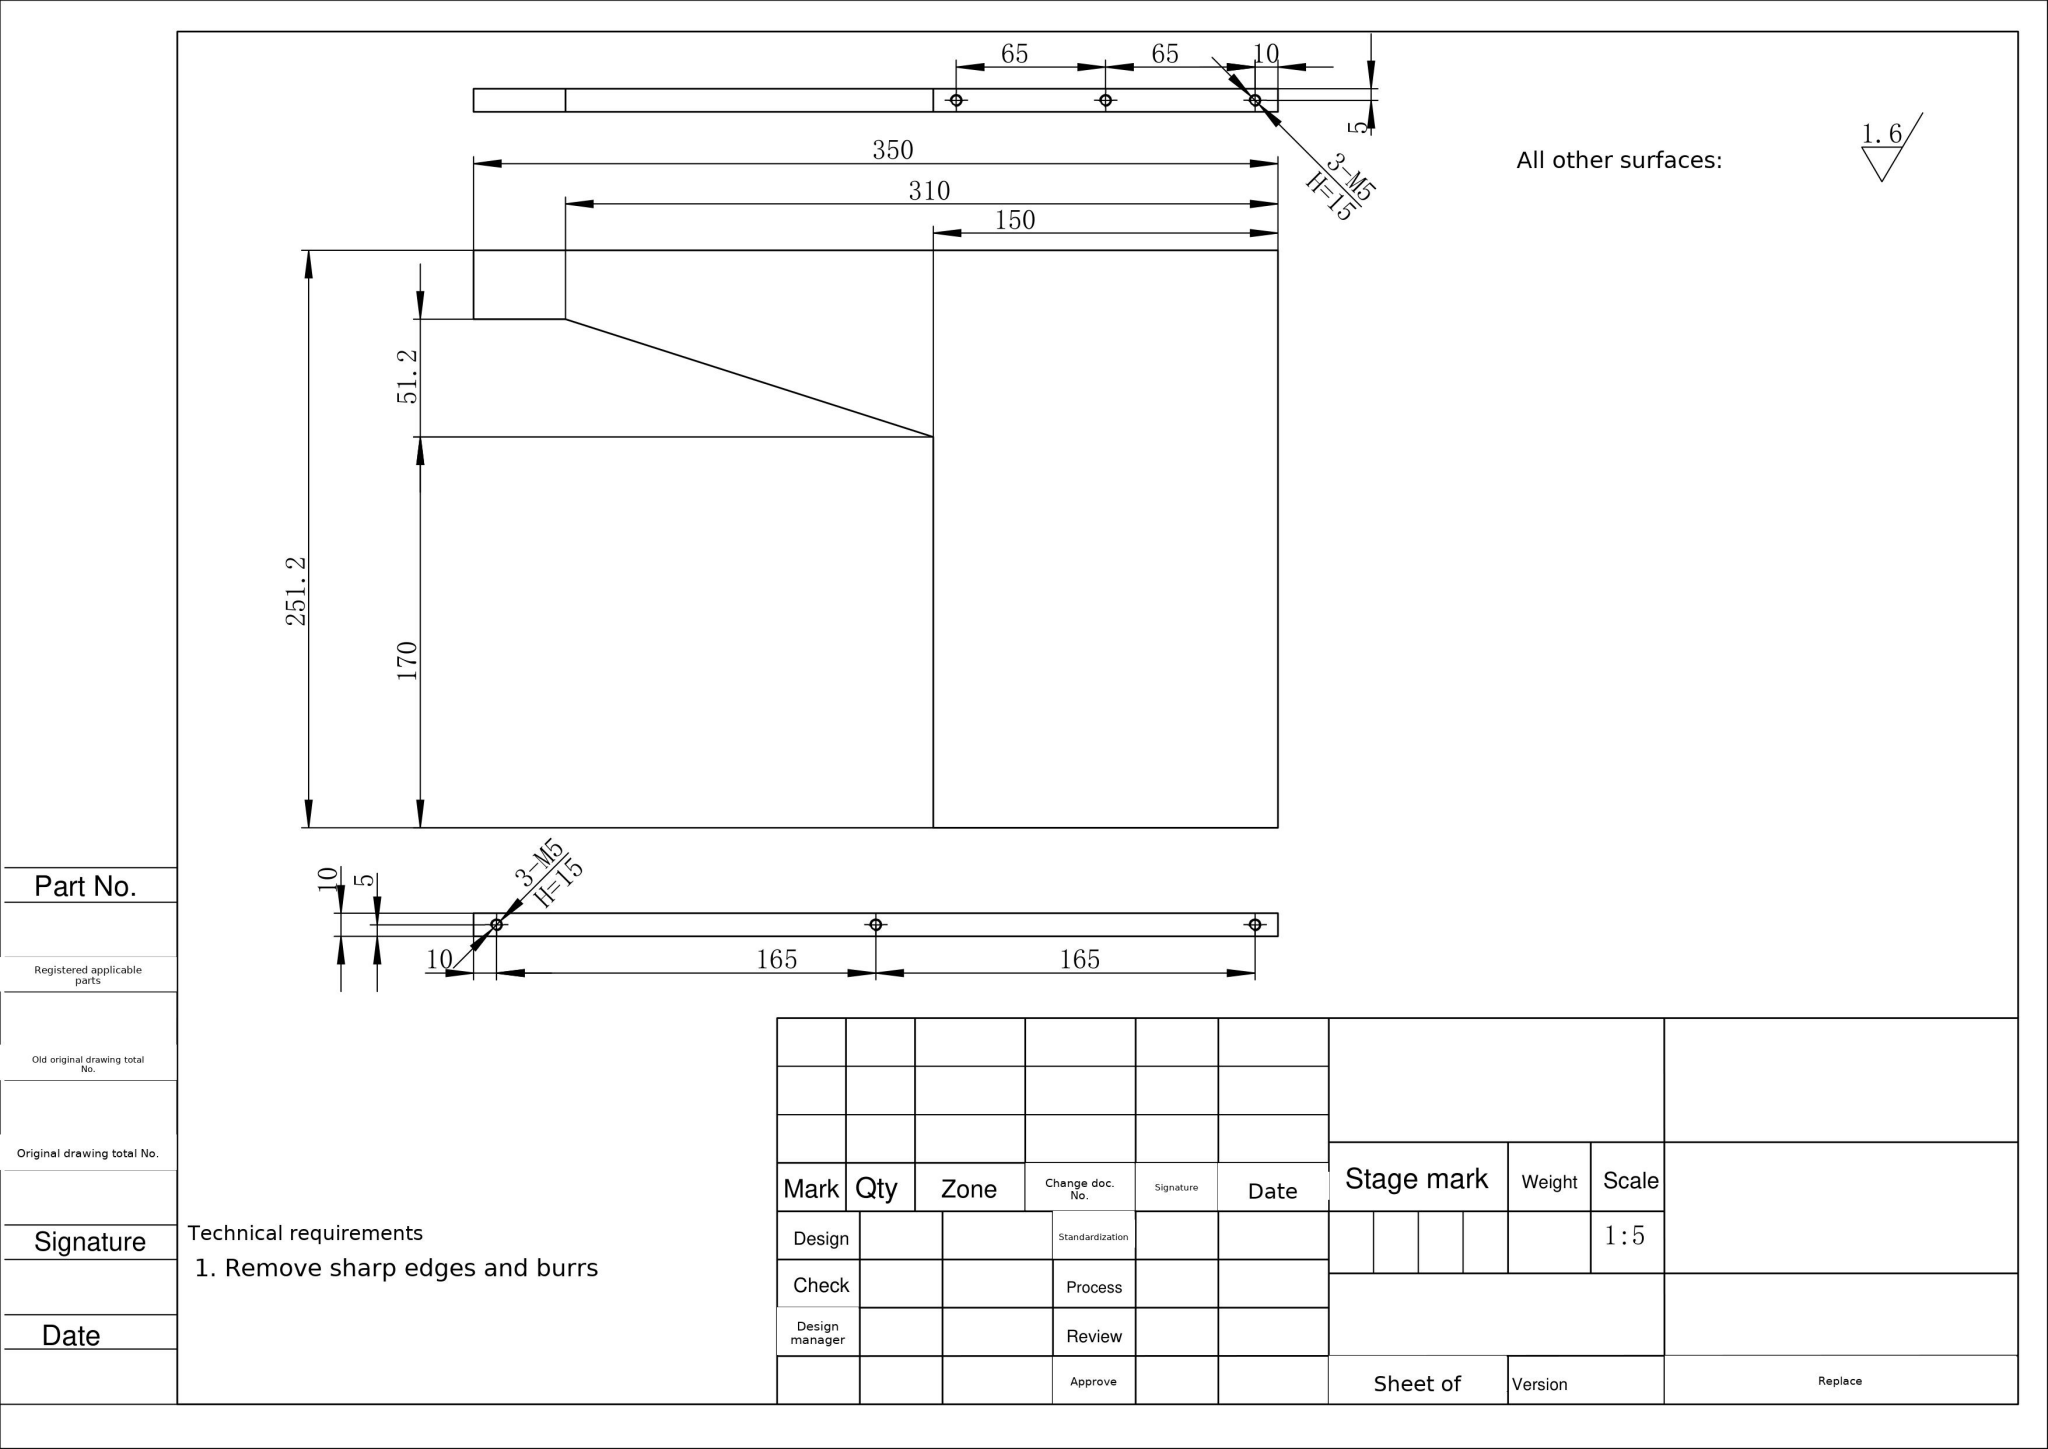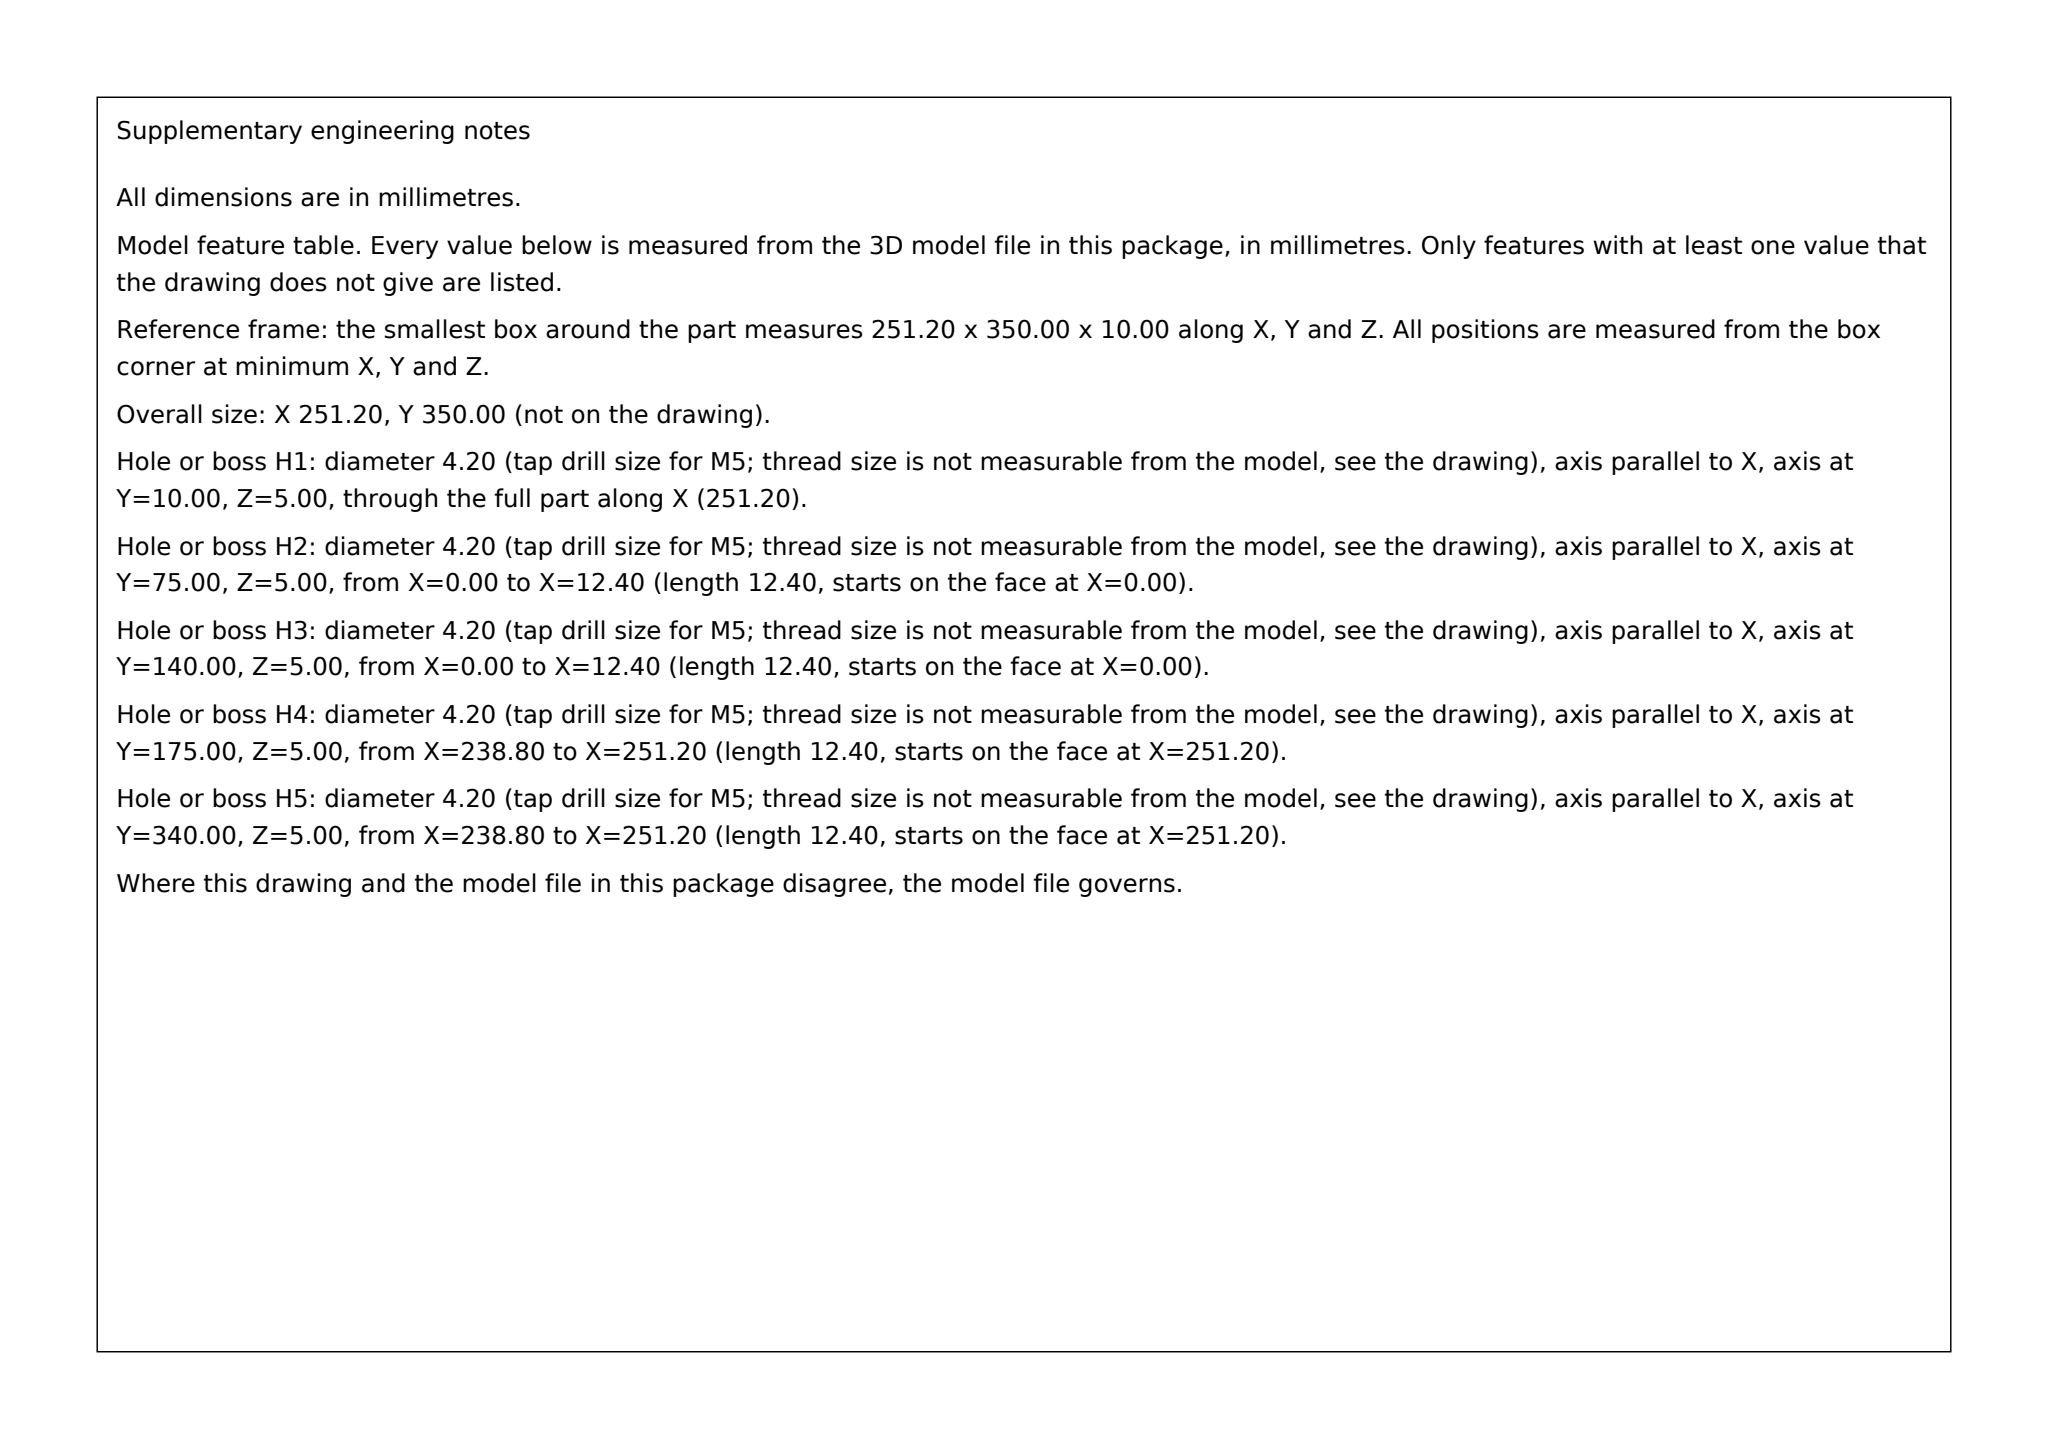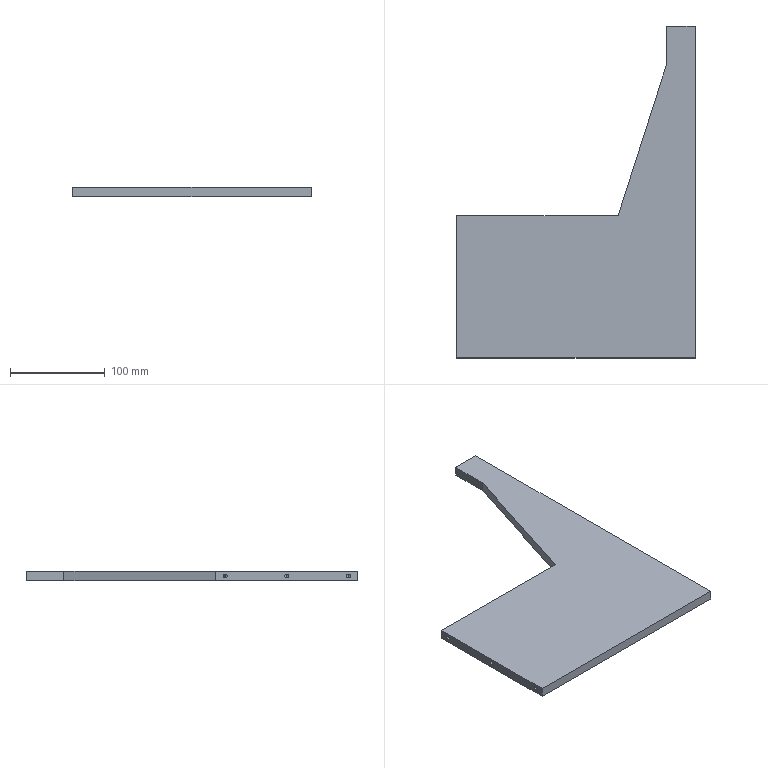Part | SolidWorks | mm | 1 solid | 33 faces | box 251.2 x 350 x 10 mm | volume 476694 mm3 | cylinder 12 | cone 12 | plane 9 | commonest cylinder face diameters 4.2 x12
build123d program:
from build123d import *

# Parameters (mm, degrees)
BOSS_EXTRUDE1_DEPTH   = 10
M5_TAPPED_HOLE1_D     = 4.2
M5_TAPPED_HOLE1_DEPTH = 12.4
M5_TAPPED_HOLE1_TIP   = 1.262
M5_TAPPED_HOLE2_D     = 4.2
M5_TAPPED_HOLE2_DEPTH = 12.4
M5_TAPPED_HOLE2_TIP   = 1.262


with BuildPart() as part:
    # Sketch1 → Boss-Extrude1 (new body)
    with BuildSketch(Plane.XY):
        Polygon((-10, 998.645), (-40, 998.645), (-40, 958.645), (-91.2, 798.645), (-261.2, 798.645), (-261.2, 648.645), (-10, 648.645), align=None)
    extrude(amount=BOSS_EXTRUDE1_DEPTH)

    # M5 Tapped Hole1
    with Locations(Plane(origin=(-10, 0, 0), x_dir=(0, 0, -1), z_dir=(1, 0, 0))):
        with Locations((-5, 658.645), (-5, 823.645), (-5, 988.645)):
            Hole(M5_TAPPED_HOLE1_D / 2, depth=M5_TAPPED_HOLE1_DEPTH)
            with Locations((0, 0, -(M5_TAPPED_HOLE1_DEPTH + M5_TAPPED_HOLE1_TIP / 2))):  # 118° drill point
                Cone(0, M5_TAPPED_HOLE1_D / 2, M5_TAPPED_HOLE1_TIP, mode=Mode.SUBTRACT)

    # M5 Tapped Hole2
    with Locations(Plane.ZY.offset(261.2)):
        with Locations((5, 788.645), (5, 723.645), (5, 658.645)):
            Hole(M5_TAPPED_HOLE2_D / 2, depth=M5_TAPPED_HOLE2_DEPTH)
            with Locations((0, 0, -(M5_TAPPED_HOLE2_DEPTH + M5_TAPPED_HOLE2_TIP / 2))):  # 118° drill point
                Cone(0, M5_TAPPED_HOLE2_D / 2, M5_TAPPED_HOLE2_TIP, mode=Mode.SUBTRACT)


solid = part.part
STEP:
#1=CARTESIAN_POINT('',(-248.8,788.645,2.9));
#2=VERTEX_POINT('',#1);
#3=CARTESIAN_POINT('',(-248.8,788.645,7.1));
#4=VERTEX_POINT('',#3);
#5=CARTESIAN_POINT('',(-248.8,788.645,5.));
#6=DIRECTION('',(-1.,0.,0.));
#7=DIRECTION('',(0.,0.,1.));
#8=AXIS2_PLACEMENT_3D('',#5,#6,#7);
#9=CIRCLE('',#8,2.1);
#10=EDGE_CURVE('',#2,#4,#9,.T.);
#11=ORIENTED_EDGE('',*,*,#10,.F.);
#12=CARTESIAN_POINT('',(-261.2,788.645,2.9));
#13=VERTEX_POINT('',#12);
#14=CARTESIAN_POINT('',(-261.2,788.645,2.9));
#15=DIRECTION('',(-1.,0.,0.));
#16=VECTOR('',#15,1000.);
#17=LINE('',#14,#16);
#18=EDGE_CURVE('',#2,#13,#17,.T.);
#19=ORIENTED_EDGE('',*,*,#18,.T.);
#20=CARTESIAN_POINT('',(-261.2,788.645,7.1));
#21=VERTEX_POINT('',#20);
#22=CARTESIAN_POINT('',(-261.2,788.645,5.));
#23=DIRECTION('',(-1.,0.,0.));
#24=DIRECTION('',(0.,0.,1.));
#25=AXIS2_PLACEMENT_3D('',#22,#23,#24);
#26=CIRCLE('',#25,2.1);
#27=EDGE_CURVE('',#13,#21,#26,.T.);
#28=ORIENTED_EDGE('',*,*,#27,.T.);
#29=CARTESIAN_POINT('',(-261.2,788.645,7.1));
#30=DIRECTION('',(-1.,0.,0.));
#31=VECTOR('',#30,1000.);
#32=LINE('',#29,#31);
#33=EDGE_CURVE('',#4,#21,#32,.T.);
#34=ORIENTED_EDGE('',*,*,#33,.F.);
#35=EDGE_LOOP('',(#11,#19,#28,#34));
#36=FACE_OUTER_BOUND('',#35,.T.);
#37=CARTESIAN_POINT('',(-261.2,788.645,5.));
#38=DIRECTION('',(-1.,0.,0.));
#39=DIRECTION('',(0.,0.,1.));
#40=AXIS2_PLACEMENT_3D('',#37,#38,#39);
#41=CYLINDRICAL_SURFACE('',#40,2.1);
#42=ADVANCED_FACE('',(#36),#41,.F.);
#43=CARTESIAN_POINT('',(-247.538,788.645,5.));
#44=VERTEX_POINT('',#43);
#45=CARTESIAN_POINT('',(-248.8,788.645,7.1));
#46=DIRECTION('',(-0.515,0.,0.8572));
#47=VECTOR('',#46,1000.);
#48=LINE('',#45,#47);
#49=EDGE_CURVE('',#44,#4,#48,.T.);
#50=ORIENTED_EDGE('',*,*,#49,.F.);
#51=CARTESIAN_POINT('',(-248.8,788.645,2.9));
#52=DIRECTION('',(-0.515,0.,-0.8572));
#53=VECTOR('',#52,1000.);
#54=LINE('',#51,#53);
#55=EDGE_CURVE('',#44,#2,#54,.T.);
#56=ORIENTED_EDGE('',*,*,#55,.T.);
#57=ORIENTED_EDGE('',*,*,#10,.T.);
#58=EDGE_LOOP('',(#50,#56,#57));
#59=FACE_OUTER_BOUND('',#58,.T.);
#60=CARTESIAN_POINT('',(-248.8,788.645,5.));
#61=DIRECTION('',(-1.,0.,0.));
#62=DIRECTION('',(0.,0.,1.));
#63=AXIS2_PLACEMENT_3D('',#60,#61,#62);
#64=CONICAL_SURFACE('',#63,2.1,1.03);
#65=ADVANCED_FACE('',(#59),#64,.F.);
#66=CARTESIAN_POINT('',(-248.8,723.645,2.9));
#67=VERTEX_POINT('',#66);
#68=CARTESIAN_POINT('',(-248.8,723.645,7.1));
#69=VERTEX_POINT('',#68);
#70=CARTESIAN_POINT('',(-248.8,723.645,5.));
#71=DIRECTION('',(-1.,0.,0.));
#72=DIRECTION('',(0.,0.,1.));
#73=AXIS2_PLACEMENT_3D('',#70,#71,#72);
#74=CIRCLE('',#73,2.1);
#75=EDGE_CURVE('',#67,#69,#74,.T.);
#76=ORIENTED_EDGE('',*,*,#75,.F.);
#77=CARTESIAN_POINT('',(-261.2,723.645,2.9));
#78=VERTEX_POINT('',#77);
#79=CARTESIAN_POINT('',(-261.2,723.645,2.9));
#80=DIRECTION('',(-1.,0.,0.));
#81=VECTOR('',#80,1000.);
#82=LINE('',#79,#81);
#83=EDGE_CURVE('',#67,#78,#82,.T.);
#84=ORIENTED_EDGE('',*,*,#83,.T.);
#85=CARTESIAN_POINT('',(-261.2,723.645,7.1));
#86=VERTEX_POINT('',#85);
#87=CARTESIAN_POINT('',(-261.2,723.645,5.));
#88=DIRECTION('',(-1.,0.,0.));
#89=DIRECTION('',(0.,0.,1.));
#90=AXIS2_PLACEMENT_3D('',#87,#88,#89);
#91=CIRCLE('',#90,2.1);
#92=EDGE_CURVE('',#78,#86,#91,.T.);
#93=ORIENTED_EDGE('',*,*,#92,.T.);
#94=CARTESIAN_POINT('',(-261.2,723.645,7.1));
#95=DIRECTION('',(-1.,0.,0.));
#96=VECTOR('',#95,1000.);
#97=LINE('',#94,#96);
#98=EDGE_CURVE('',#69,#86,#97,.T.);
#99=ORIENTED_EDGE('',*,*,#98,.F.);
#100=EDGE_LOOP('',(#76,#84,#93,#99));
#101=FACE_OUTER_BOUND('',#100,.T.);
#102=CARTESIAN_POINT('',(-261.2,723.645,5.));
#103=DIRECTION('',(-1.,0.,0.));
#104=DIRECTION('',(0.,0.,1.));
#105=AXIS2_PLACEMENT_3D('',#102,#103,#104);
#106=CYLINDRICAL_SURFACE('',#105,2.1);
#107=ADVANCED_FACE('',(#101),#106,.F.);
#108=CARTESIAN_POINT('',(-247.538,723.645,5.));
#109=VERTEX_POINT('',#108);
#110=CARTESIAN_POINT('',(-248.8,723.645,7.1));
#111=DIRECTION('',(-0.515,0.,0.8572));
#112=VECTOR('',#111,1000.);
#113=LINE('',#110,#112);
#114=EDGE_CURVE('',#109,#69,#113,.T.);
#115=ORIENTED_EDGE('',*,*,#114,.F.);
#116=CARTESIAN_POINT('',(-248.8,723.645,2.9));
#117=DIRECTION('',(-0.515,0.,-0.8572));
#118=VECTOR('',#117,1000.);
#119=LINE('',#116,#118);
#120=EDGE_CURVE('',#109,#67,#119,.T.);
#121=ORIENTED_EDGE('',*,*,#120,.T.);
#122=ORIENTED_EDGE('',*,*,#75,.T.);
#123=EDGE_LOOP('',(#115,#121,#122));
#124=FACE_OUTER_BOUND('',#123,.T.);
#125=CARTESIAN_POINT('',(-248.8,723.645,5.));
#126=DIRECTION('',(-1.,0.,0.));
#127=DIRECTION('',(0.,0.,1.));
#128=AXIS2_PLACEMENT_3D('',#125,#126,#127);
#129=CONICAL_SURFACE('',#128,2.1,1.03);
#130=ADVANCED_FACE('',(#124),#129,.F.);
#131=CARTESIAN_POINT('',(-248.8,658.645,2.9));
#132=VERTEX_POINT('',#131);
#133=CARTESIAN_POINT('',(-248.8,658.645,7.1));
#134=VERTEX_POINT('',#133);
#135=CARTESIAN_POINT('',(-248.8,658.645,5.));
#136=DIRECTION('',(-1.,0.,0.));
#137=DIRECTION('',(0.,0.,1.));
#138=AXIS2_PLACEMENT_3D('',#135,#136,#137);
#139=CIRCLE('',#138,2.1);
#140=EDGE_CURVE('',#132,#134,#139,.T.);
#141=ORIENTED_EDGE('',*,*,#140,.F.);
#142=CARTESIAN_POINT('',(-261.2,658.645,2.9));
#143=VERTEX_POINT('',#142);
#144=CARTESIAN_POINT('',(-261.2,658.645,2.9));
#145=DIRECTION('',(-1.,0.,0.));
#146=VECTOR('',#145,1000.);
#147=LINE('',#144,#146);
#148=EDGE_CURVE('',#132,#143,#147,.T.);
#149=ORIENTED_EDGE('',*,*,#148,.T.);
#150=CARTESIAN_POINT('',(-261.2,658.645,7.1));
#151=VERTEX_POINT('',#150);
#152=CARTESIAN_POINT('',(-261.2,658.645,5.));
#153=DIRECTION('',(-1.,0.,0.));
#154=DIRECTION('',(0.,0.,1.));
#155=AXIS2_PLACEMENT_3D('',#152,#153,#154);
#156=CIRCLE('',#155,2.1);
#157=EDGE_CURVE('',#143,#151,#156,.T.);
#158=ORIENTED_EDGE('',*,*,#157,.T.);
#159=CARTESIAN_POINT('',(-261.2,658.645,7.1));
#160=DIRECTION('',(-1.,0.,0.));
#161=VECTOR('',#160,1000.);
#162=LINE('',#159,#161);
#163=EDGE_CURVE('',#134,#151,#162,.T.);
#164=ORIENTED_EDGE('',*,*,#163,.F.);
#165=EDGE_LOOP('',(#141,#149,#158,#164));
#166=FACE_OUTER_BOUND('',#165,.T.);
#167=CARTESIAN_POINT('',(-261.2,658.645,5.));
#168=DIRECTION('',(-1.,0.,0.));
#169=DIRECTION('',(0.,0.,1.));
#170=AXIS2_PLACEMENT_3D('',#167,#168,#169);
#171=CYLINDRICAL_SURFACE('',#170,2.1);
#172=ADVANCED_FACE('',(#166),#171,.F.);
#173=CARTESIAN_POINT('',(-247.538,658.645,5.));
#174=VERTEX_POINT('',#173);
#175=CARTESIAN_POINT('',(-248.8,658.645,7.1));
#176=DIRECTION('',(-0.515,0.,0.8572));
#177=VECTOR('',#176,1000.);
#178=LINE('',#175,#177);
#179=EDGE_CURVE('',#174,#134,#178,.T.);
#180=ORIENTED_EDGE('',*,*,#179,.F.);
#181=CARTESIAN_POINT('',(-248.8,658.645,2.9));
#182=DIRECTION('',(-0.515,0.,-0.8572));
#183=VECTOR('',#182,1000.);
#184=LINE('',#181,#183);
#185=EDGE_CURVE('',#174,#132,#184,.T.);
#186=ORIENTED_EDGE('',*,*,#185,.T.);
#187=ORIENTED_EDGE('',*,*,#140,.T.);
#188=EDGE_LOOP('',(#180,#186,#187));
#189=FACE_OUTER_BOUND('',#188,.T.);
#190=CARTESIAN_POINT('',(-248.8,658.645,5.));
#191=DIRECTION('',(-1.,0.,0.));
#192=DIRECTION('',(0.,0.,1.));
#193=AXIS2_PLACEMENT_3D('',#190,#191,#192);
#194=CONICAL_SURFACE('',#193,2.1,1.03);
#195=ADVANCED_FACE('',(#189),#194,.F.);
#196=CARTESIAN_POINT('',(-22.4,658.645,7.1));
#197=VERTEX_POINT('',#196);
#198=CARTESIAN_POINT('',(-22.4,658.645,2.9));
#199=VERTEX_POINT('',#198);
#200=CARTESIAN_POINT('',(-22.4,658.645,5.));
#201=DIRECTION('',(1.,0.,0.));
#202=DIRECTION('',(0.,0.,-1.));
#203=AXIS2_PLACEMENT_3D('',#200,#201,#202);
#204=CIRCLE('',#203,2.1);
#205=EDGE_CURVE('',#197,#199,#204,.T.);
#206=ORIENTED_EDGE('',*,*,#205,.F.);
#207=CARTESIAN_POINT('',(-10.,658.645,7.1));
#208=VERTEX_POINT('',#207);
#209=CARTESIAN_POINT('',(-10.,658.645,7.1));
#210=DIRECTION('',(1.,0.,0.));
#211=VECTOR('',#210,1000.);
#212=LINE('',#209,#211);
#213=EDGE_CURVE('',#197,#208,#212,.T.);
#214=ORIENTED_EDGE('',*,*,#213,.T.);
#215=CARTESIAN_POINT('',(-10.,658.645,2.9));
#216=VERTEX_POINT('',#215);
#217=CARTESIAN_POINT('',(-10.,658.645,5.));
#218=DIRECTION('',(1.,0.,0.));
#219=DIRECTION('',(0.,0.,-1.));
#220=AXIS2_PLACEMENT_3D('',#217,#218,#219);
#221=CIRCLE('',#220,2.1);
#222=EDGE_CURVE('',#208,#216,#221,.T.);
#223=ORIENTED_EDGE('',*,*,#222,.T.);
#224=CARTESIAN_POINT('',(-10.,658.645,2.9));
#225=DIRECTION('',(1.,0.,0.));
#226=VECTOR('',#225,1000.);
#227=LINE('',#224,#226);
#228=EDGE_CURVE('',#199,#216,#227,.T.);
#229=ORIENTED_EDGE('',*,*,#228,.F.);
#230=EDGE_LOOP('',(#206,#214,#223,#229));
#231=FACE_OUTER_BOUND('',#230,.T.);
#232=CARTESIAN_POINT('',(-10.,658.645,5.));
#233=DIRECTION('',(1.,0.,0.));
#234=DIRECTION('',(0.,0.,-1.));
#235=AXIS2_PLACEMENT_3D('',#232,#233,#234);
#236=CYLINDRICAL_SURFACE('',#235,2.1);
#237=ADVANCED_FACE('',(#231),#236,.F.);
#238=CARTESIAN_POINT('',(-23.662,658.645,5.));
#239=VERTEX_POINT('',#238);
#240=CARTESIAN_POINT('',(-22.4,658.645,2.9));
#241=DIRECTION('',(0.515,0.,-0.8572));
#242=VECTOR('',#241,1000.);
#243=LINE('',#240,#242);
#244=EDGE_CURVE('',#239,#199,#243,.T.);
#245=ORIENTED_EDGE('',*,*,#244,.F.);
#246=CARTESIAN_POINT('',(-22.4,658.645,7.1));
#247=DIRECTION('',(0.515,0.,0.8572));
#248=VECTOR('',#247,1000.);
#249=LINE('',#246,#248);
#250=EDGE_CURVE('',#239,#197,#249,.T.);
#251=ORIENTED_EDGE('',*,*,#250,.T.);
#252=ORIENTED_EDGE('',*,*,#205,.T.);
#253=EDGE_LOOP('',(#245,#251,#252));
#254=FACE_OUTER_BOUND('',#253,.T.);
#255=CARTESIAN_POINT('',(-22.4,658.645,5.));
#256=DIRECTION('',(1.,0.,0.));
#257=DIRECTION('',(0.,0.,-1.));
#258=AXIS2_PLACEMENT_3D('',#255,#256,#257);
#259=CONICAL_SURFACE('',#258,2.1,1.03);
#260=ADVANCED_FACE('',(#254),#259,.F.);
#261=CARTESIAN_POINT('',(-22.4,823.645,7.1));
#262=VERTEX_POINT('',#261);
#263=CARTESIAN_POINT('',(-22.4,823.645,2.9));
#264=VERTEX_POINT('',#263);
#265=CARTESIAN_POINT('',(-22.4,823.645,5.));
#266=DIRECTION('',(1.,0.,0.));
#267=DIRECTION('',(0.,0.,-1.));
#268=AXIS2_PLACEMENT_3D('',#265,#266,#267);
#269=CIRCLE('',#268,2.1);
#270=EDGE_CURVE('',#262,#264,#269,.T.);
#271=ORIENTED_EDGE('',*,*,#270,.F.);
#272=CARTESIAN_POINT('',(-10.,823.645,7.1));
#273=VERTEX_POINT('',#272);
#274=CARTESIAN_POINT('',(-10.,823.645,7.1));
#275=DIRECTION('',(1.,0.,0.));
#276=VECTOR('',#275,1000.);
#277=LINE('',#274,#276);
#278=EDGE_CURVE('',#262,#273,#277,.T.);
#279=ORIENTED_EDGE('',*,*,#278,.T.);
#280=CARTESIAN_POINT('',(-10.,823.645,2.9));
#281=VERTEX_POINT('',#280);
#282=CARTESIAN_POINT('',(-10.,823.645,5.));
#283=DIRECTION('',(1.,0.,0.));
#284=DIRECTION('',(0.,0.,-1.));
#285=AXIS2_PLACEMENT_3D('',#282,#283,#284);
#286=CIRCLE('',#285,2.1);
#287=EDGE_CURVE('',#273,#281,#286,.T.);
#288=ORIENTED_EDGE('',*,*,#287,.T.);
#289=CARTESIAN_POINT('',(-10.,823.645,2.9));
#290=DIRECTION('',(1.,0.,0.));
#291=VECTOR('',#290,1000.);
#292=LINE('',#289,#291);
#293=EDGE_CURVE('',#264,#281,#292,.T.);
#294=ORIENTED_EDGE('',*,*,#293,.F.);
#295=EDGE_LOOP('',(#271,#279,#288,#294));
#296=FACE_OUTER_BOUND('',#295,.T.);
#297=CARTESIAN_POINT('',(-10.,823.645,5.));
#298=DIRECTION('',(1.,0.,0.));
#299=DIRECTION('',(0.,0.,-1.));
#300=AXIS2_PLACEMENT_3D('',#297,#298,#299);
#301=CYLINDRICAL_SURFACE('',#300,2.1);
#302=ADVANCED_FACE('',(#296),#301,.F.);
#303=CARTESIAN_POINT('',(-23.662,823.645,5.));
#304=VERTEX_POINT('',#303);
#305=CARTESIAN_POINT('',(-22.4,823.645,2.9));
#306=DIRECTION('',(0.515,0.,-0.8572));
#307=VECTOR('',#306,1000.);
#308=LINE('',#305,#307);
#309=EDGE_CURVE('',#304,#264,#308,.T.);
#310=ORIENTED_EDGE('',*,*,#309,.F.);
#311=CARTESIAN_POINT('',(-22.4,823.645,7.1));
#312=DIRECTION('',(0.515,0.,0.8572));
#313=VECTOR('',#312,1000.);
#314=LINE('',#311,#313);
#315=EDGE_CURVE('',#304,#262,#314,.T.);
#316=ORIENTED_EDGE('',*,*,#315,.T.);
#317=ORIENTED_EDGE('',*,*,#270,.T.);
#318=EDGE_LOOP('',(#310,#316,#317));
#319=FACE_OUTER_BOUND('',#318,.T.);
#320=CARTESIAN_POINT('',(-22.4,823.645,5.));
#321=DIRECTION('',(1.,0.,0.));
#322=DIRECTION('',(0.,0.,-1.));
#323=AXIS2_PLACEMENT_3D('',#320,#321,#322);
#324=CONICAL_SURFACE('',#323,2.1,1.03);
#325=ADVANCED_FACE('',(#319),#324,.F.);
#326=CARTESIAN_POINT('',(-22.4,988.645,7.1));
#327=VERTEX_POINT('',#326);
#328=CARTESIAN_POINT('',(-22.4,988.645,2.9));
#329=VERTEX_POINT('',#328);
#330=CARTESIAN_POINT('',(-22.4,988.645,5.));
#331=DIRECTION('',(1.,0.,0.));
#332=DIRECTION('',(0.,0.,-1.));
#333=AXIS2_PLACEMENT_3D('',#330,#331,#332);
#334=CIRCLE('',#333,2.1);
#335=EDGE_CURVE('',#327,#329,#334,.T.);
#336=ORIENTED_EDGE('',*,*,#335,.F.);
#337=CARTESIAN_POINT('',(-10.,988.645,7.1));
#338=VERTEX_POINT('',#337);
#339=CARTESIAN_POINT('',(-10.,988.645,7.1));
#340=DIRECTION('',(1.,0.,0.));
#341=VECTOR('',#340,1000.);
#342=LINE('',#339,#341);
#343=EDGE_CURVE('',#327,#338,#342,.T.);
#344=ORIENTED_EDGE('',*,*,#343,.T.);
#345=CARTESIAN_POINT('',(-10.,988.645,2.9));
#346=VERTEX_POINT('',#345);
#347=CARTESIAN_POINT('',(-10.,988.645,5.));
#348=DIRECTION('',(1.,0.,0.));
#349=DIRECTION('',(0.,0.,-1.));
#350=AXIS2_PLACEMENT_3D('',#347,#348,#349);
#351=CIRCLE('',#350,2.1);
#352=EDGE_CURVE('',#338,#346,#351,.T.);
#353=ORIENTED_EDGE('',*,*,#352,.T.);
#354=CARTESIAN_POINT('',(-10.,988.645,2.9));
#355=DIRECTION('',(1.,0.,0.));
#356=VECTOR('',#355,1000.);
#357=LINE('',#354,#356);
#358=EDGE_CURVE('',#329,#346,#357,.T.);
#359=ORIENTED_EDGE('',*,*,#358,.F.);
#360=EDGE_LOOP('',(#336,#344,#353,#359));
#361=FACE_OUTER_BOUND('',#360,.T.);
#362=CARTESIAN_POINT('',(-10.,988.645,5.));
#363=DIRECTION('',(1.,0.,0.));
#364=DIRECTION('',(0.,0.,-1.));
#365=AXIS2_PLACEMENT_3D('',#362,#363,#364);
#366=CYLINDRICAL_SURFACE('',#365,2.1);
#367=ADVANCED_FACE('',(#361),#366,.F.);
#368=CARTESIAN_POINT('',(-23.662,988.645,5.));
#369=VERTEX_POINT('',#368);
#370=CARTESIAN_POINT('',(-22.4,988.645,2.9));
#371=DIRECTION('',(0.515,0.,-0.8572));
#372=VECTOR('',#371,1000.);
#373=LINE('',#370,#372);
#374=EDGE_CURVE('',#369,#329,#373,.T.);
#375=ORIENTED_EDGE('',*,*,#374,.F.);
#376=CARTESIAN_POINT('',(-22.4,988.645,7.1));
#377=DIRECTION('',(0.515,0.,0.8572));
#378=VECTOR('',#377,1000.);
#379=LINE('',#376,#378);
#380=EDGE_CURVE('',#369,#327,#379,.T.);
#381=ORIENTED_EDGE('',*,*,#380,.T.);
#382=ORIENTED_EDGE('',*,*,#335,.T.);
#383=EDGE_LOOP('',(#375,#381,#382));
#384=FACE_OUTER_BOUND('',#383,.T.);
#385=CARTESIAN_POINT('',(-22.4,988.645,5.));
#386=DIRECTION('',(1.,0.,0.));
#387=DIRECTION('',(0.,0.,-1.));
#388=AXIS2_PLACEMENT_3D('',#385,#386,#387);
#389=CONICAL_SURFACE('',#388,2.1,1.03);
#390=ADVANCED_FACE('',(#384),#389,.F.);
#391=CARTESIAN_POINT('',(-10.,658.645,5.));
#392=DIRECTION('',(1.,0.,0.));
#393=DIRECTION('',(0.,0.,-1.));
#394=AXIS2_PLACEMENT_3D('',#391,#392,#393);
#395=CIRCLE('',#394,2.1);
#396=EDGE_CURVE('',#216,#208,#395,.T.);
#397=ORIENTED_EDGE('',*,*,#396,.F.);
#398=ORIENTED_EDGE('',*,*,#222,.F.);
#399=EDGE_LOOP('',(#397,#398));
#400=FACE_BOUND('',#399,.T.);
#401=CARTESIAN_POINT('',(-10.,823.645,5.));
#402=DIRECTION('',(1.,0.,0.));
#403=DIRECTION('',(0.,0.,-1.));
#404=AXIS2_PLACEMENT_3D('',#401,#402,#403);
#405=CIRCLE('',#404,2.1);
#406=EDGE_CURVE('',#281,#273,#405,.T.);
#407=ORIENTED_EDGE('',*,*,#406,.F.);
#408=ORIENTED_EDGE('',*,*,#287,.F.);
#409=EDGE_LOOP('',(#407,#408));
#410=FACE_BOUND('',#409,.T.);
#411=CARTESIAN_POINT('',(-10.,988.645,5.));
#412=DIRECTION('',(1.,0.,0.));
#413=DIRECTION('',(0.,0.,-1.));
#414=AXIS2_PLACEMENT_3D('',#411,#412,#413);
#415=CIRCLE('',#414,2.1);
#416=EDGE_CURVE('',#346,#338,#415,.T.);
#417=ORIENTED_EDGE('',*,*,#416,.F.);
#418=ORIENTED_EDGE('',*,*,#352,.F.);
#419=EDGE_LOOP('',(#417,#418));
#420=FACE_BOUND('',#419,.T.);
#421=CARTESIAN_POINT('',(-10.,648.645,0.));
#422=VERTEX_POINT('',#421);
#423=CARTESIAN_POINT('',(-10.,998.645,0.));
#424=VERTEX_POINT('',#423);
#425=CARTESIAN_POINT('',(-10.,648.645,0.));
#426=DIRECTION('',(0.,1.,0.));
#427=VECTOR('',#426,1000.);
#428=LINE('',#425,#427);
#429=EDGE_CURVE('',#422,#424,#428,.T.);
#430=ORIENTED_EDGE('',*,*,#429,.T.);
#431=CARTESIAN_POINT('',(-10.,998.645,10.));
#432=VERTEX_POINT('',#431);
#433=CARTESIAN_POINT('',(-10.,998.645,10.));
#434=DIRECTION('',(0.,0.,-1.));
#435=VECTOR('',#434,1000.);
#436=LINE('',#433,#435);
#437=EDGE_CURVE('',#432,#424,#436,.T.);
#438=ORIENTED_EDGE('',*,*,#437,.F.);
#439=CARTESIAN_POINT('',(-10.,648.645,10.));
#440=VERTEX_POINT('',#439);
#441=CARTESIAN_POINT('',(-10.,648.645,10.));
#442=DIRECTION('',(0.,1.,0.));
#443=VECTOR('',#442,1000.);
#444=LINE('',#441,#443);
#445=EDGE_CURVE('',#440,#432,#444,.T.);
#446=ORIENTED_EDGE('',*,*,#445,.F.);
#447=CARTESIAN_POINT('',(-10.,648.645,10.));
#448=DIRECTION('',(0.,0.,-1.));
#449=VECTOR('',#448,1000.);
#450=LINE('',#447,#449);
#451=EDGE_CURVE('',#440,#422,#450,.T.);
#452=ORIENTED_EDGE('',*,*,#451,.T.);
#453=EDGE_LOOP('',(#430,#438,#446,#452));
#454=FACE_OUTER_BOUND('',#453,.T.);
#455=CARTESIAN_POINT('',(-10.,648.645,10.));
#456=DIRECTION('',(-1.,0.,0.));
#457=DIRECTION('',(0.,0.,1.));
#458=AXIS2_PLACEMENT_3D('',#455,#456,#457);
#459=PLANE('',#458);
#460=ADVANCED_FACE('',(#400,#410,#420,#454),#459,.F.);
#461=CARTESIAN_POINT('',(-40.,998.645,0.));
#462=VERTEX_POINT('',#461);
#463=CARTESIAN_POINT('',(-10.,998.645,0.));
#464=DIRECTION('',(-1.,0.,0.));
#465=VECTOR('',#464,1000.);
#466=LINE('',#463,#465);
#467=EDGE_CURVE('',#424,#462,#466,.T.);
#468=ORIENTED_EDGE('',*,*,#467,.T.);
#469=CARTESIAN_POINT('',(-40.,998.645,10.));
#470=VERTEX_POINT('',#469);
#471=CARTESIAN_POINT('',(-40.,998.645,10.));
#472=DIRECTION('',(0.,0.,-1.));
#473=VECTOR('',#472,1000.);
#474=LINE('',#471,#473);
#475=EDGE_CURVE('',#470,#462,#474,.T.);
#476=ORIENTED_EDGE('',*,*,#475,.F.);
#477=CARTESIAN_POINT('',(-10.,998.645,10.));
#478=DIRECTION('',(-1.,0.,0.));
#479=VECTOR('',#478,1000.);
#480=LINE('',#477,#479);
#481=EDGE_CURVE('',#432,#470,#480,.T.);
#482=ORIENTED_EDGE('',*,*,#481,.F.);
#483=ORIENTED_EDGE('',*,*,#437,.T.);
#484=EDGE_LOOP('',(#468,#476,#482,#483));
#485=FACE_OUTER_BOUND('',#484,.T.);
#486=CARTESIAN_POINT('',(-10.,998.645,10.));
#487=DIRECTION('',(-0.,-1.,0.));
#488=DIRECTION('',(1.,-0.,0.));
#489=AXIS2_PLACEMENT_3D('',#486,#487,#488);
#490=PLANE('',#489);
#491=ADVANCED_FACE('',(#485),#490,.F.);
#492=CARTESIAN_POINT('',(-40.,958.645,0.));
#493=VERTEX_POINT('',#492);
#494=CARTESIAN_POINT('',(-40.,998.645,0.));
#495=DIRECTION('',(0.,-1.,0.));
#496=VECTOR('',#495,1000.);
#497=LINE('',#494,#496);
#498=EDGE_CURVE('',#462,#493,#497,.T.);
#499=ORIENTED_EDGE('',*,*,#498,.T.);
#500=CARTESIAN_POINT('',(-40.,958.645,10.));
#501=VERTEX_POINT('',#500);
#502=CARTESIAN_POINT('',(-40.,958.645,10.));
#503=DIRECTION('',(0.,0.,-1.));
#504=VECTOR('',#503,1000.);
#505=LINE('',#502,#504);
#506=EDGE_CURVE('',#501,#493,#505,.T.);
#507=ORIENTED_EDGE('',*,*,#506,.F.);
#508=CARTESIAN_POINT('',(-40.,998.645,10.));
#509=DIRECTION('',(0.,-1.,0.));
#510=VECTOR('',#509,1000.);
#511=LINE('',#508,#510);
#512=EDGE_CURVE('',#470,#501,#511,.T.);
#513=ORIENTED_EDGE('',*,*,#512,.F.);
#514=ORIENTED_EDGE('',*,*,#475,.T.);
#515=EDGE_LOOP('',(#499,#507,#513,#514));
#516=FACE_OUTER_BOUND('',#515,.T.);
#517=CARTESIAN_POINT('',(-40.,998.645,10.));
#518=DIRECTION('',(1.,0.,0.));
#519=DIRECTION('',(-0.,1.,0.));
#520=AXIS2_PLACEMENT_3D('',#517,#518,#519);
#521=PLANE('',#520);
#522=ADVANCED_FACE('',(#516),#521,.F.);
#523=CARTESIAN_POINT('',(-91.2,798.645,0.));
#524=VERTEX_POINT('',#523);
#525=CARTESIAN_POINT('',(-40.,958.645,0.));
#526=DIRECTION('',(-0.3048,-0.9524,0.));
#527=VECTOR('',#526,1000.);
#528=LINE('',#525,#527);
#529=EDGE_CURVE('',#493,#524,#528,.T.);
#530=ORIENTED_EDGE('',*,*,#529,.T.);
#531=CARTESIAN_POINT('',(-91.2,798.645,10.));
#532=VERTEX_POINT('',#531);
#533=CARTESIAN_POINT('',(-91.2,798.645,10.));
#534=DIRECTION('',(0.,0.,-1.));
#535=VECTOR('',#534,1000.);
#536=LINE('',#533,#535);
#537=EDGE_CURVE('',#532,#524,#536,.T.);
#538=ORIENTED_EDGE('',*,*,#537,.F.);
#539=CARTESIAN_POINT('',(-40.,958.645,10.));
#540=DIRECTION('',(-0.3048,-0.9524,0.));
#541=VECTOR('',#540,1000.);
#542=LINE('',#539,#541);
#543=EDGE_CURVE('',#501,#532,#542,.T.);
#544=ORIENTED_EDGE('',*,*,#543,.F.);
#545=ORIENTED_EDGE('',*,*,#506,.T.);
#546=EDGE_LOOP('',(#530,#538,#544,#545));
#547=FACE_OUTER_BOUND('',#546,.T.);
#548=CARTESIAN_POINT('',(-40.,958.645,10.));
#549=DIRECTION('',(0.9524,-0.3048,0.));
#550=DIRECTION('',(0.3048,0.9524,0.));
#551=AXIS2_PLACEMENT_3D('',#548,#549,#550);
#552=PLANE('',#551);
#553=ADVANCED_FACE('',(#547),#552,.F.);
#554=CARTESIAN_POINT('',(-261.2,798.645,0.));
#555=VERTEX_POINT('',#554);
#556=CARTESIAN_POINT('',(-91.2,798.645,0.));
#557=DIRECTION('',(-1.,0.,0.));
#558=VECTOR('',#557,1000.);
#559=LINE('',#556,#558);
#560=EDGE_CURVE('',#524,#555,#559,.T.);
#561=ORIENTED_EDGE('',*,*,#560,.T.);
#562=CARTESIAN_POINT('',(-261.2,798.645,10.));
#563=VERTEX_POINT('',#562);
#564=CARTESIAN_POINT('',(-261.2,798.645,10.));
#565=DIRECTION('',(0.,0.,-1.));
#566=VECTOR('',#565,1000.);
#567=LINE('',#564,#566);
#568=EDGE_CURVE('',#563,#555,#567,.T.);
#569=ORIENTED_EDGE('',*,*,#568,.F.);
#570=CARTESIAN_POINT('',(-91.2,798.645,10.));
#571=DIRECTION('',(-1.,0.,0.));
#572=VECTOR('',#571,1000.);
#573=LINE('',#570,#572);
#574=EDGE_CURVE('',#532,#563,#573,.T.);
#575=ORIENTED_EDGE('',*,*,#574,.F.);
#576=ORIENTED_EDGE('',*,*,#537,.T.);
#577=EDGE_LOOP('',(#561,#569,#575,#576));
#578=FACE_OUTER_BOUND('',#577,.T.);
#579=CARTESIAN_POINT('',(-91.2,798.645,10.));
#580=DIRECTION('',(0.,-1.,0.));
#581=DIRECTION('',(0.,0.,-1.));
#582=AXIS2_PLACEMENT_3D('',#579,#580,#581);
#583=PLANE('',#582);
#584=ADVANCED_FACE('',(#578),#583,.F.);
#585=CARTESIAN_POINT('',(-261.2,788.645,5.));
#586=DIRECTION('',(-1.,0.,0.));
#587=DIRECTION('',(0.,0.,1.));
#588=AXIS2_PLACEMENT_3D('',#585,#586,#587);
#589=CIRCLE('',#588,2.1);
#590=EDGE_CURVE('',#21,#13,#589,.T.);
#591=ORIENTED_EDGE('',*,*,#590,.F.);
#592=ORIENTED_EDGE('',*,*,#27,.F.);
#593=EDGE_LOOP('',(#591,#592));
#594=FACE_BOUND('',#593,.T.);
#595=CARTESIAN_POINT('',(-261.2,723.645,5.));
#596=DIRECTION('',(-1.,0.,0.));
#597=DIRECTION('',(0.,0.,1.));
#598=AXIS2_PLACEMENT_3D('',#595,#596,#597);
#599=CIRCLE('',#598,2.1);
#600=EDGE_CURVE('',#86,#78,#599,.T.);
#601=ORIENTED_EDGE('',*,*,#600,.F.);
#602=ORIENTED_EDGE('',*,*,#92,.F.);
#603=EDGE_LOOP('',(#601,#602));
#604=FACE_BOUND('',#603,.T.);
#605=CARTESIAN_POINT('',(-261.2,658.645,5.));
#606=DIRECTION('',(-1.,0.,0.));
#607=DIRECTION('',(0.,0.,1.));
#608=AXIS2_PLACEMENT_3D('',#605,#606,#607);
#609=CIRCLE('',#608,2.1);
#610=EDGE_CURVE('',#151,#143,#609,.T.);
#611=ORIENTED_EDGE('',*,*,#610,.F.);
#612=ORIENTED_EDGE('',*,*,#157,.F.);
#613=EDGE_LOOP('',(#611,#612));
#614=FACE_BOUND('',#613,.T.);
#615=CARTESIAN_POINT('',(-261.2,648.645,0.));
#616=VERTEX_POINT('',#615);
#617=CARTESIAN_POINT('',(-261.2,798.645,0.));
#618=DIRECTION('',(0.,-1.,0.));
#619=VECTOR('',#618,1000.);
#620=LINE('',#617,#619);
#621=EDGE_CURVE('',#555,#616,#620,.T.);
#622=ORIENTED_EDGE('',*,*,#621,.T.);
#623=CARTESIAN_POINT('',(-261.2,648.645,10.));
#624=VERTEX_POINT('',#623);
#625=CARTESIAN_POINT('',(-261.2,648.645,10.));
#626=DIRECTION('',(0.,0.,-1.));
#627=VECTOR('',#626,1000.);
#628=LINE('',#625,#627);
#629=EDGE_CURVE('',#624,#616,#628,.T.);
#630=ORIENTED_EDGE('',*,*,#629,.F.);
#631=CARTESIAN_POINT('',(-261.2,798.645,10.));
#632=DIRECTION('',(0.,-1.,0.));
#633=VECTOR('',#632,1000.);
#634=LINE('',#631,#633);
#635=EDGE_CURVE('',#563,#624,#634,.T.);
#636=ORIENTED_EDGE('',*,*,#635,.F.);
#637=ORIENTED_EDGE('',*,*,#568,.T.);
#638=EDGE_LOOP('',(#622,#630,#636,#637));
#639=FACE_OUTER_BOUND('',#638,.T.);
#640=CARTESIAN_POINT('',(-261.2,798.645,10.));
#641=DIRECTION('',(1.,0.,0.));
#642=DIRECTION('',(0.,0.,-1.));
#643=AXIS2_PLACEMENT_3D('',#640,#641,#642);
#644=PLANE('',#643);
#645=ADVANCED_FACE('',(#594,#604,#614,#639),#644,.F.);
#646=CARTESIAN_POINT('',(-261.2,648.645,0.));
#647=DIRECTION('',(1.,0.,0.));
#648=VECTOR('',#647,1000.);
#649=LINE('',#646,#648);
#650=EDGE_CURVE('',#616,#422,#649,.T.);
#651=ORIENTED_EDGE('',*,*,#650,.T.);
#652=ORIENTED_EDGE('',*,*,#451,.F.);
#653=CARTESIAN_POINT('',(-261.2,648.645,10.));
#654=DIRECTION('',(1.,0.,0.));
#655=VECTOR('',#654,1000.);
#656=LINE('',#653,#655);
#657=EDGE_CURVE('',#624,#440,#656,.T.);
#658=ORIENTED_EDGE('',*,*,#657,.F.);
#659=ORIENTED_EDGE('',*,*,#629,.T.);
#660=EDGE_LOOP('',(#651,#652,#658,#659));
#661=FACE_OUTER_BOUND('',#660,.T.);
#662=CARTESIAN_POINT('',(-261.2,648.645,10.));
#663=DIRECTION('',(0.,1.,0.));
#664=DIRECTION('',(0.,0.,1.));
#665=AXIS2_PLACEMENT_3D('',#662,#663,#664);
#666=PLANE('',#665);
#667=ADVANCED_FACE('',(#661),#666,.F.);
#668=ORIENTED_EDGE('',*,*,#445,.T.);
#669=ORIENTED_EDGE('',*,*,#481,.T.);
#670=ORIENTED_EDGE('',*,*,#512,.T.);
#671=ORIENTED_EDGE('',*,*,#543,.T.);
#672=ORIENTED_EDGE('',*,*,#574,.T.);
#673=ORIENTED_EDGE('',*,*,#635,.T.);
#674=ORIENTED_EDGE('',*,*,#657,.T.);
#675=EDGE_LOOP('',(#668,#669,#670,#671,#672,#673,#674));
#676=FACE_OUTER_BOUND('',#675,.T.);
#677=CARTESIAN_POINT('',(0.,0.,10.));
#678=DIRECTION('',(0.,0.,1.));
#679=DIRECTION('',(1.,0.,0.));
#680=AXIS2_PLACEMENT_3D('',#677,#678,#679);
#681=PLANE('',#680);
#682=ADVANCED_FACE('',(#676),#681,.T.);
#683=ORIENTED_EDGE('',*,*,#429,.F.);
#684=ORIENTED_EDGE('',*,*,#650,.F.);
#685=ORIENTED_EDGE('',*,*,#621,.F.);
#686=ORIENTED_EDGE('',*,*,#560,.F.);
#687=ORIENTED_EDGE('',*,*,#529,.F.);
#688=ORIENTED_EDGE('',*,*,#498,.F.);
#689=ORIENTED_EDGE('',*,*,#467,.F.);
#690=EDGE_LOOP('',(#683,#684,#685,#686,#687,#688,#689));
#691=FACE_OUTER_BOUND('',#690,.T.);
#692=CARTESIAN_POINT('',(0.,0.,0.));
#693=DIRECTION('',(0.,0.,1.));
#694=DIRECTION('',(1.,0.,0.));
#695=AXIS2_PLACEMENT_3D('',#692,#693,#694);
#696=PLANE('',#695);
#697=ADVANCED_FACE('',(#691),#696,.F.);
#698=ORIENTED_EDGE('',*,*,#380,.F.);
#699=ORIENTED_EDGE('',*,*,#374,.T.);
#700=CARTESIAN_POINT('',(-22.4,988.645,5.));
#701=DIRECTION('',(1.,0.,0.));
#702=DIRECTION('',(0.,0.,-1.));
#703=AXIS2_PLACEMENT_3D('',#700,#701,#702);
#704=CIRCLE('',#703,2.1);
#705=EDGE_CURVE('',#329,#327,#704,.T.);
#706=ORIENTED_EDGE('',*,*,#705,.T.);
#707=EDGE_LOOP('',(#698,#699,#706));
#708=FACE_OUTER_BOUND('',#707,.T.);
#709=CARTESIAN_POINT('',(-22.4,988.645,5.));
#710=DIRECTION('',(1.,0.,0.));
#711=DIRECTION('',(0.,0.,-1.));
#712=AXIS2_PLACEMENT_3D('',#709,#710,#711);
#713=CONICAL_SURFACE('',#712,2.1,1.03);
#714=ADVANCED_FACE('',(#708),#713,.F.);
#715=ORIENTED_EDGE('',*,*,#343,.F.);
#716=ORIENTED_EDGE('',*,*,#705,.F.);
#717=ORIENTED_EDGE('',*,*,#358,.T.);
#718=ORIENTED_EDGE('',*,*,#416,.T.);
#719=EDGE_LOOP('',(#715,#716,#717,#718));
#720=FACE_OUTER_BOUND('',#719,.T.);
#721=CARTESIAN_POINT('',(-10.,988.645,5.));
#722=DIRECTION('',(1.,0.,0.));
#723=DIRECTION('',(0.,0.,-1.));
#724=AXIS2_PLACEMENT_3D('',#721,#722,#723);
#725=CYLINDRICAL_SURFACE('',#724,2.1);
#726=ADVANCED_FACE('',(#720),#725,.F.);
#727=ORIENTED_EDGE('',*,*,#315,.F.);
#728=ORIENTED_EDGE('',*,*,#309,.T.);
#729=CARTESIAN_POINT('',(-22.4,823.645,5.));
#730=DIRECTION('',(1.,0.,0.));
#731=DIRECTION('',(0.,0.,-1.));
#732=AXIS2_PLACEMENT_3D('',#729,#730,#731);
#733=CIRCLE('',#732,2.1);
#734=EDGE_CURVE('',#264,#262,#733,.T.);
#735=ORIENTED_EDGE('',*,*,#734,.T.);
#736=EDGE_LOOP('',(#727,#728,#735));
#737=FACE_OUTER_BOUND('',#736,.T.);
#738=CARTESIAN_POINT('',(-22.4,823.645,5.));
#739=DIRECTION('',(1.,0.,0.));
#740=DIRECTION('',(0.,0.,-1.));
#741=AXIS2_PLACEMENT_3D('',#738,#739,#740);
#742=CONICAL_SURFACE('',#741,2.1,1.03);
#743=ADVANCED_FACE('',(#737),#742,.F.);
#744=ORIENTED_EDGE('',*,*,#278,.F.);
#745=ORIENTED_EDGE('',*,*,#734,.F.);
#746=ORIENTED_EDGE('',*,*,#293,.T.);
#747=ORIENTED_EDGE('',*,*,#406,.T.);
#748=EDGE_LOOP('',(#744,#745,#746,#747));
#749=FACE_OUTER_BOUND('',#748,.T.);
#750=CARTESIAN_POINT('',(-10.,823.645,5.));
#751=DIRECTION('',(1.,0.,0.));
#752=DIRECTION('',(0.,0.,-1.));
#753=AXIS2_PLACEMENT_3D('',#750,#751,#752);
#754=CYLINDRICAL_SURFACE('',#753,2.1);
#755=ADVANCED_FACE('',(#749),#754,.F.);
#756=ORIENTED_EDGE('',*,*,#250,.F.);
#757=ORIENTED_EDGE('',*,*,#244,.T.);
#758=CARTESIAN_POINT('',(-22.4,658.645,5.));
#759=DIRECTION('',(1.,0.,0.));
#760=DIRECTION('',(0.,0.,-1.));
#761=AXIS2_PLACEMENT_3D('',#758,#759,#760);
#762=CIRCLE('',#761,2.1);
#763=EDGE_CURVE('',#199,#197,#762,.T.);
#764=ORIENTED_EDGE('',*,*,#763,.T.);
#765=EDGE_LOOP('',(#756,#757,#764));
#766=FACE_OUTER_BOUND('',#765,.T.);
#767=CARTESIAN_POINT('',(-22.4,658.645,5.));
#768=DIRECTION('',(1.,0.,0.));
#769=DIRECTION('',(0.,0.,-1.));
#770=AXIS2_PLACEMENT_3D('',#767,#768,#769);
#771=CONICAL_SURFACE('',#770,2.1,1.03);
#772=ADVANCED_FACE('',(#766),#771,.F.);
#773=ORIENTED_EDGE('',*,*,#213,.F.);
#774=ORIENTED_EDGE('',*,*,#763,.F.);
#775=ORIENTED_EDGE('',*,*,#228,.T.);
#776=ORIENTED_EDGE('',*,*,#396,.T.);
#777=EDGE_LOOP('',(#773,#774,#775,#776));
#778=FACE_OUTER_BOUND('',#777,.T.);
#779=CARTESIAN_POINT('',(-10.,658.645,5.));
#780=DIRECTION('',(1.,0.,0.));
#781=DIRECTION('',(0.,0.,-1.));
#782=AXIS2_PLACEMENT_3D('',#779,#780,#781);
#783=CYLINDRICAL_SURFACE('',#782,2.1);
#784=ADVANCED_FACE('',(#778),#783,.F.);
#785=ORIENTED_EDGE('',*,*,#185,.F.);
#786=ORIENTED_EDGE('',*,*,#179,.T.);
#787=CARTESIAN_POINT('',(-248.8,658.645,5.));
#788=DIRECTION('',(-1.,0.,0.));
#789=DIRECTION('',(0.,0.,1.));
#790=AXIS2_PLACEMENT_3D('',#787,#788,#789);
#791=CIRCLE('',#790,2.1);
#792=EDGE_CURVE('',#134,#132,#791,.T.);
#793=ORIENTED_EDGE('',*,*,#792,.T.);
#794=EDGE_LOOP('',(#785,#786,#793));
#795=FACE_OUTER_BOUND('',#794,.T.);
#796=CARTESIAN_POINT('',(-248.8,658.645,5.));
#797=DIRECTION('',(-1.,0.,0.));
#798=DIRECTION('',(0.,0.,1.));
#799=AXIS2_PLACEMENT_3D('',#796,#797,#798);
#800=CONICAL_SURFACE('',#799,2.1,1.03);
#801=ADVANCED_FACE('',(#795),#800,.F.);
#802=ORIENTED_EDGE('',*,*,#148,.F.);
#803=ORIENTED_EDGE('',*,*,#792,.F.);
#804=ORIENTED_EDGE('',*,*,#163,.T.);
#805=ORIENTED_EDGE('',*,*,#610,.T.);
#806=EDGE_LOOP('',(#802,#803,#804,#805));
#807=FACE_OUTER_BOUND('',#806,.T.);
#808=CARTESIAN_POINT('',(-261.2,658.645,5.));
#809=DIRECTION('',(-1.,0.,0.));
#810=DIRECTION('',(0.,0.,1.));
#811=AXIS2_PLACEMENT_3D('',#808,#809,#810);
#812=CYLINDRICAL_SURFACE('',#811,2.1);
#813=ADVANCED_FACE('',(#807),#812,.F.);
#814=ORIENTED_EDGE('',*,*,#120,.F.);
#815=ORIENTED_EDGE('',*,*,#114,.T.);
#816=CARTESIAN_POINT('',(-248.8,723.645,5.));
#817=DIRECTION('',(-1.,0.,0.));
#818=DIRECTION('',(0.,0.,1.));
#819=AXIS2_PLACEMENT_3D('',#816,#817,#818);
#820=CIRCLE('',#819,2.1);
#821=EDGE_CURVE('',#69,#67,#820,.T.);
#822=ORIENTED_EDGE('',*,*,#821,.T.);
#823=EDGE_LOOP('',(#814,#815,#822));
#824=FACE_OUTER_BOUND('',#823,.T.);
#825=CARTESIAN_POINT('',(-248.8,723.645,5.));
#826=DIRECTION('',(-1.,0.,0.));
#827=DIRECTION('',(0.,0.,1.));
#828=AXIS2_PLACEMENT_3D('',#825,#826,#827);
#829=CONICAL_SURFACE('',#828,2.1,1.03);
#830=ADVANCED_FACE('',(#824),#829,.F.);
#831=ORIENTED_EDGE('',*,*,#83,.F.);
#832=ORIENTED_EDGE('',*,*,#821,.F.);
#833=ORIENTED_EDGE('',*,*,#98,.T.);
#834=ORIENTED_EDGE('',*,*,#600,.T.);
#835=EDGE_LOOP('',(#831,#832,#833,#834));
#836=FACE_OUTER_BOUND('',#835,.T.);
#837=CARTESIAN_POINT('',(-261.2,723.645,5.));
#838=DIRECTION('',(-1.,0.,0.));
#839=DIRECTION('',(0.,0.,1.));
#840=AXIS2_PLACEMENT_3D('',#837,#838,#839);
#841=CYLINDRICAL_SURFACE('',#840,2.1);
#842=ADVANCED_FACE('',(#836),#841,.F.);
#843=ORIENTED_EDGE('',*,*,#55,.F.);
#844=ORIENTED_EDGE('',*,*,#49,.T.);
#845=CARTESIAN_POINT('',(-248.8,788.645,5.));
#846=DIRECTION('',(-1.,0.,0.));
#847=DIRECTION('',(0.,0.,1.));
#848=AXIS2_PLACEMENT_3D('',#845,#846,#847);
#849=CIRCLE('',#848,2.1);
#850=EDGE_CURVE('',#4,#2,#849,.T.);
#851=ORIENTED_EDGE('',*,*,#850,.T.);
#852=EDGE_LOOP('',(#843,#844,#851));
#853=FACE_OUTER_BOUND('',#852,.T.);
#854=CARTESIAN_POINT('',(-248.8,788.645,5.));
#855=DIRECTION('',(-1.,0.,0.));
#856=DIRECTION('',(0.,0.,1.));
#857=AXIS2_PLACEMENT_3D('',#854,#855,#856);
#858=CONICAL_SURFACE('',#857,2.1,1.03);
#859=ADVANCED_FACE('',(#853),#858,.F.);
#860=ORIENTED_EDGE('',*,*,#18,.F.);
#861=ORIENTED_EDGE('',*,*,#850,.F.);
#862=ORIENTED_EDGE('',*,*,#33,.T.);
#863=ORIENTED_EDGE('',*,*,#590,.T.);
#864=EDGE_LOOP('',(#860,#861,#862,#863));
#865=FACE_OUTER_BOUND('',#864,.T.);
#866=CARTESIAN_POINT('',(-261.2,788.645,5.));
#867=DIRECTION('',(-1.,0.,0.));
#868=DIRECTION('',(0.,0.,1.));
#869=AXIS2_PLACEMENT_3D('',#866,#867,#868);
#870=CYLINDRICAL_SURFACE('',#869,2.1);
#871=ADVANCED_FACE('',(#865),#870,.F.);
#872=CLOSED_SHELL('',(#42,#65,#107,#130,#172,#195,#237,#260,#302,#325,#367,#390,#460,#491,#522,#553,#584,#645,#667,#682,#697,#714,#726,#743,#755,#772,#784,#801,#813,#830,#842,#859,#871));
#873=MANIFOLD_SOLID_BREP('',#872);
#874=CARTESIAN_POINT('',(0.,0.,0.));
#875=DIRECTION('',(0.,0.,1.));
#876=DIRECTION('',(1.,0.,0.));
#877=AXIS2_PLACEMENT_3D('',#874,#875,#876);
#878=(LENGTH_UNIT()NAMED_UNIT(*)SI_UNIT(.MILLI.,.METRE.));
#879=UNCERTAINTY_MEASURE_WITH_UNIT(LENGTH_MEASURE(0.00001),#878,'','');
#880=(NAMED_UNIT(*)PLANE_ANGLE_UNIT()SI_UNIT($,.RADIAN.));
#881=(NAMED_UNIT(*)SI_UNIT($,.STERADIAN.)SOLID_ANGLE_UNIT());
#882=(GEOMETRIC_REPRESENTATION_CONTEXT(3)GLOBAL_UNCERTAINTY_ASSIGNED_CONTEXT((#879))GLOBAL_UNIT_ASSIGNED_CONTEXT((#878,#880,#881))REPRESENTATION_CONTEXT('',''));
#883=ADVANCED_BREP_SHAPE_REPRESENTATION('',(#873,#877),#882);